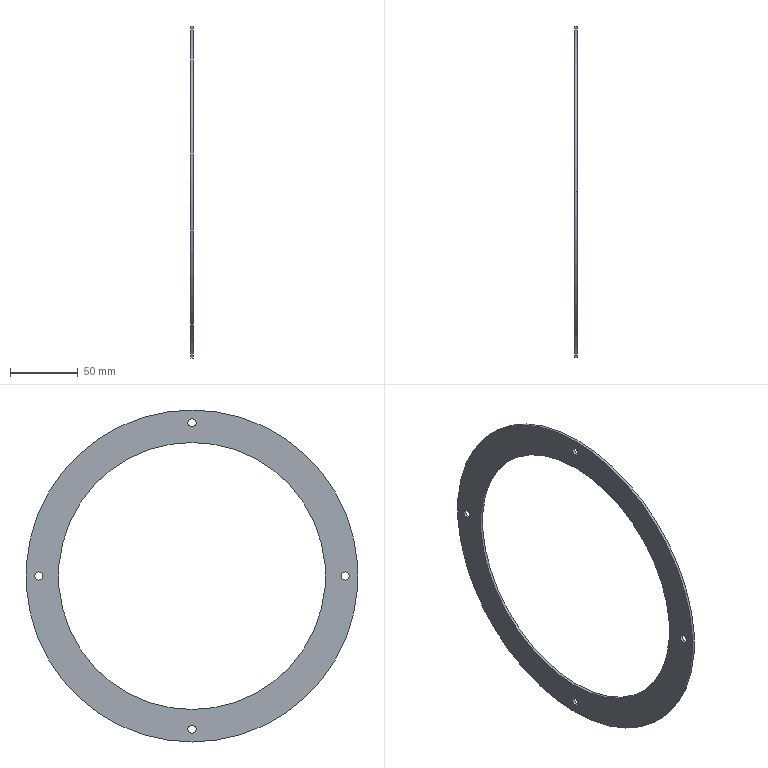Component | SolidWorks | RoundBaffle-1 | 1 solid | 14 faces | box 2 x 245 x 245 mm | volume 33100 mm3 | cylinder 12 | plane 2 | commonest cylinder face diameters 6 x8 197 x2 245 x2
build123d program:
from build123d import *

# Parameters (mm, degrees)
SKETCH1_R           = 122.5
SKETCH1_R_2         = 98.5
BOSS_EXTRUDE1_DEPTH = 2
SKETCH2_R           = 3
CUT_EXTRUDE1_DEPTH  = 10
CIRPATTERN1_COUNT   = 4


with BuildPart() as part:
    # Sketch1 → Boss-Extrude1 (new body)
    with BuildSketch(Plane.XY):
        Circle(SKETCH1_R)
        Circle(SKETCH1_R_2, mode=Mode.SUBTRACT)
    extrude(amount=BOSS_EXTRUDE1_DEPTH)

    # Sketch2 → Cut-Extrude1 (cut)
    with BuildSketch(Plane.XY.offset(2)):
        with Locations((0, 113)):
            Circle(SKETCH2_R)
    cut_extrude1 = extrude(amount=-CUT_EXTRUDE1_DEPTH, mode=Mode.SUBTRACT)

    # CirPattern1: Cut-Extrude1 ×4 about axis
    cirpattern1_axis = Axis((0, 0, 0), (0, 0, 1))
    for i in range(1, CIRPATTERN1_COUNT):
        add(cut_extrude1.rotate(cirpattern1_axis, i * 360 / CIRPATTERN1_COUNT), mode=Mode.SUBTRACT)


solid = part.part

# Placed as in the assembly
solid = solid.moved(Location((-292.55, -77.904, 57.481), (0, 90, 0)))
STEP:
#1=COLOUR_RGB('',0.7922,0.8196,0.9333);
#2=FILL_AREA_STYLE_COLOUR('',#1);
#3=FILL_AREA_STYLE('',(#2));
#4=SURFACE_STYLE_FILL_AREA(#3);
#5=SURFACE_SIDE_STYLE('',(#4));
#6=SURFACE_STYLE_USAGE(.BOTH.,#5);
#7=PRESENTATION_STYLE_ASSIGNMENT((#6));
#8=CARTESIAN_POINT('',(-11.439,-3.067,6.594));
#9=VERTEX_POINT('',#8);
#10=CARTESIAN_POINT('',(-11.439,-3.067,6.83));
#11=VERTEX_POINT('',#10);
#12=CARTESIAN_POINT('',(-11.439,-3.067,6.712));
#13=DIRECTION('',(-1.,0.,0.));
#14=DIRECTION('',(0.,0.,1.));
#15=AXIS2_PLACEMENT_3D('',#12,#13,#14);
#16=CIRCLE('',#15,0.1181);
#17=EDGE_CURVE('',#9,#11,#16,.T.);
#18=ORIENTED_EDGE('',*,*,#17,.F.);
#19=CARTESIAN_POINT('',(-11.518,-3.067,6.594));
#20=VERTEX_POINT('',#19);
#21=CARTESIAN_POINT('',(-11.124,-3.067,6.594));
#22=DIRECTION('',(-1.,0.,0.));
#23=VECTOR('',#22,39.37);
#24=LINE('',#21,#23);
#25=EDGE_CURVE('',#9,#20,#24,.T.);
#26=ORIENTED_EDGE('',*,*,#25,.T.);
#27=CARTESIAN_POINT('',(-11.518,-3.067,6.83));
#28=VERTEX_POINT('',#27);
#29=CARTESIAN_POINT('',(-11.518,-3.067,6.712));
#30=DIRECTION('',(-1.,0.,0.));
#31=DIRECTION('',(0.,-1.,0.));
#32=AXIS2_PLACEMENT_3D('',#29,#30,#31);
#33=CIRCLE('',#32,0.1181);
#34=EDGE_CURVE('',#20,#28,#33,.T.);
#35=ORIENTED_EDGE('',*,*,#34,.T.);
#36=CARTESIAN_POINT('',(-11.124,-3.067,6.83));
#37=DIRECTION('',(-1.,0.,0.));
#38=VECTOR('',#37,39.37);
#39=LINE('',#36,#38);
#40=EDGE_CURVE('',#11,#28,#39,.T.);
#41=ORIENTED_EDGE('',*,*,#40,.F.);
#42=EDGE_LOOP('',(#18,#26,#35,#41));
#43=FACE_OUTER_BOUND('',#42,.T.);
#44=CARTESIAN_POINT('',(-11.124,-3.067,6.712));
#45=DIRECTION('',(-1.,0.,0.));
#46=DIRECTION('',(0.,0.,1.));
#47=AXIS2_PLACEMENT_3D('',#44,#45,#46);
#48=CYLINDRICAL_SURFACE('',#47,0.1181);
#49=ADVANCED_FACE('',(#43),#48,.F.);
#50=CARTESIAN_POINT('',(-11.439,-7.516,2.145));
#51=VERTEX_POINT('',#50);
#52=CARTESIAN_POINT('',(-11.439,-7.516,2.381));
#53=VERTEX_POINT('',#52);
#54=CARTESIAN_POINT('',(-11.439,-7.516,2.263));
#55=DIRECTION('',(-1.,0.,0.));
#56=DIRECTION('',(0.,0.,1.));
#57=AXIS2_PLACEMENT_3D('',#54,#55,#56);
#58=CIRCLE('',#57,0.1181);
#59=EDGE_CURVE('',#51,#53,#58,.T.);
#60=ORIENTED_EDGE('',*,*,#59,.F.);
#61=CARTESIAN_POINT('',(-11.518,-7.516,2.145));
#62=VERTEX_POINT('',#61);
#63=CARTESIAN_POINT('',(-11.124,-7.516,2.145));
#64=DIRECTION('',(-1.,0.,0.));
#65=VECTOR('',#64,39.37);
#66=LINE('',#63,#65);
#67=EDGE_CURVE('',#51,#62,#66,.T.);
#68=ORIENTED_EDGE('',*,*,#67,.T.);
#69=CARTESIAN_POINT('',(-11.518,-7.516,2.381));
#70=VERTEX_POINT('',#69);
#71=CARTESIAN_POINT('',(-11.518,-7.516,2.263));
#72=DIRECTION('',(-1.,0.,0.));
#73=DIRECTION('',(0.,0.,-1.));
#74=AXIS2_PLACEMENT_3D('',#71,#72,#73);
#75=CIRCLE('',#74,0.1181);
#76=EDGE_CURVE('',#62,#70,#75,.T.);
#77=ORIENTED_EDGE('',*,*,#76,.T.);
#78=CARTESIAN_POINT('',(-11.124,-7.516,2.381));
#79=DIRECTION('',(-1.,0.,0.));
#80=VECTOR('',#79,39.37);
#81=LINE('',#78,#80);
#82=EDGE_CURVE('',#53,#70,#81,.T.);
#83=ORIENTED_EDGE('',*,*,#82,.F.);
#84=EDGE_LOOP('',(#60,#68,#77,#83));
#85=FACE_OUTER_BOUND('',#84,.T.);
#86=CARTESIAN_POINT('',(-11.124,-7.516,2.263));
#87=DIRECTION('',(-1.,0.,0.));
#88=DIRECTION('',(0.,0.,1.));
#89=AXIS2_PLACEMENT_3D('',#86,#87,#88);
#90=CYLINDRICAL_SURFACE('',#89,0.1181);
#91=ADVANCED_FACE('',(#85),#90,.F.);
#92=CARTESIAN_POINT('',(-11.439,-3.067,-2.304));
#93=VERTEX_POINT('',#92);
#94=CARTESIAN_POINT('',(-11.439,-3.067,-2.068));
#95=VERTEX_POINT('',#94);
#96=CARTESIAN_POINT('',(-11.439,-3.067,-2.186));
#97=DIRECTION('',(-1.,0.,0.));
#98=DIRECTION('',(0.,0.,1.));
#99=AXIS2_PLACEMENT_3D('',#96,#97,#98);
#100=CIRCLE('',#99,0.1181);
#101=EDGE_CURVE('',#93,#95,#100,.T.);
#102=ORIENTED_EDGE('',*,*,#101,.F.);
#103=CARTESIAN_POINT('',(-11.518,-3.067,-2.304));
#104=VERTEX_POINT('',#103);
#105=CARTESIAN_POINT('',(-11.124,-3.067,-2.304));
#106=DIRECTION('',(-1.,0.,0.));
#107=VECTOR('',#106,39.37);
#108=LINE('',#105,#107);
#109=EDGE_CURVE('',#93,#104,#108,.T.);
#110=ORIENTED_EDGE('',*,*,#109,.T.);
#111=CARTESIAN_POINT('',(-11.518,-3.067,-2.068));
#112=VERTEX_POINT('',#111);
#113=CARTESIAN_POINT('',(-11.518,-3.067,-2.186));
#114=DIRECTION('',(-1.,0.,0.));
#115=DIRECTION('',(0.,1.,-0.));
#116=AXIS2_PLACEMENT_3D('',#113,#114,#115);
#117=CIRCLE('',#116,0.1181);
#118=EDGE_CURVE('',#104,#112,#117,.T.);
#119=ORIENTED_EDGE('',*,*,#118,.T.);
#120=CARTESIAN_POINT('',(-11.124,-3.067,-2.068));
#121=DIRECTION('',(-1.,0.,0.));
#122=VECTOR('',#121,39.37);
#123=LINE('',#120,#122);
#124=EDGE_CURVE('',#95,#112,#123,.T.);
#125=ORIENTED_EDGE('',*,*,#124,.F.);
#126=EDGE_LOOP('',(#102,#110,#119,#125));
#127=FACE_OUTER_BOUND('',#126,.T.);
#128=CARTESIAN_POINT('',(-11.124,-3.067,-2.186));
#129=DIRECTION('',(-1.,0.,0.));
#130=DIRECTION('',(0.,0.,1.));
#131=AXIS2_PLACEMENT_3D('',#128,#129,#130);
#132=CYLINDRICAL_SURFACE('',#131,0.1181);
#133=ADVANCED_FACE('',(#127),#132,.F.);
#134=CARTESIAN_POINT('',(-11.439,1.382,2.145));
#135=VERTEX_POINT('',#134);
#136=CARTESIAN_POINT('',(-11.439,1.382,2.381));
#137=VERTEX_POINT('',#136);
#138=CARTESIAN_POINT('',(-11.439,1.382,2.263));
#139=DIRECTION('',(-1.,0.,0.));
#140=DIRECTION('',(0.,0.,1.));
#141=AXIS2_PLACEMENT_3D('',#138,#139,#140);
#142=CIRCLE('',#141,0.1181);
#143=EDGE_CURVE('',#135,#137,#142,.T.);
#144=ORIENTED_EDGE('',*,*,#143,.F.);
#145=CARTESIAN_POINT('',(-11.518,1.382,2.145));
#146=VERTEX_POINT('',#145);
#147=CARTESIAN_POINT('',(-11.124,1.382,2.145));
#148=DIRECTION('',(-1.,0.,0.));
#149=VECTOR('',#148,39.37);
#150=LINE('',#147,#149);
#151=EDGE_CURVE('',#135,#146,#150,.T.);
#152=ORIENTED_EDGE('',*,*,#151,.T.);
#153=CARTESIAN_POINT('',(-11.518,1.382,2.381));
#154=VERTEX_POINT('',#153);
#155=CARTESIAN_POINT('',(-11.518,1.382,2.263));
#156=DIRECTION('',(-1.,0.,0.));
#157=DIRECTION('',(0.,0.,1.));
#158=AXIS2_PLACEMENT_3D('',#155,#156,#157);
#159=CIRCLE('',#158,0.1181);
#160=EDGE_CURVE('',#146,#154,#159,.T.);
#161=ORIENTED_EDGE('',*,*,#160,.T.);
#162=CARTESIAN_POINT('',(-11.124,1.382,2.381));
#163=DIRECTION('',(-1.,0.,0.));
#164=VECTOR('',#163,39.37);
#165=LINE('',#162,#164);
#166=EDGE_CURVE('',#137,#154,#165,.T.);
#167=ORIENTED_EDGE('',*,*,#166,.F.);
#168=EDGE_LOOP('',(#144,#152,#161,#167));
#169=FACE_OUTER_BOUND('',#168,.T.);
#170=CARTESIAN_POINT('',(-11.124,1.382,2.263));
#171=DIRECTION('',(-1.,0.,0.));
#172=DIRECTION('',(0.,0.,1.));
#173=AXIS2_PLACEMENT_3D('',#170,#171,#172);
#174=CYLINDRICAL_SURFACE('',#173,0.1181);
#175=ADVANCED_FACE('',(#169),#174,.F.);
#176=CARTESIAN_POINT('',(-11.518,-3.067,-1.615));
#177=VERTEX_POINT('',#176);
#178=CARTESIAN_POINT('',(-11.518,-3.067,6.141));
#179=VERTEX_POINT('',#178);
#180=CARTESIAN_POINT('',(-11.518,-3.067,2.263));
#181=DIRECTION('',(-1.,0.,0.));
#182=DIRECTION('',(0.,0.,1.));
#183=AXIS2_PLACEMENT_3D('',#180,#181,#182);
#184=CIRCLE('',#183,3.878);
#185=EDGE_CURVE('',#177,#179,#184,.T.);
#186=ORIENTED_EDGE('',*,*,#185,.T.);
#187=CARTESIAN_POINT('',(-11.439,-3.067,6.141));
#188=VERTEX_POINT('',#187);
#189=CARTESIAN_POINT('',(-11.518,-3.067,6.141));
#190=DIRECTION('',(1.,0.,0.));
#191=VECTOR('',#190,39.37);
#192=LINE('',#189,#191);
#193=EDGE_CURVE('',#179,#188,#192,.T.);
#194=ORIENTED_EDGE('',*,*,#193,.T.);
#195=CARTESIAN_POINT('',(-11.439,-3.067,-1.615));
#196=VERTEX_POINT('',#195);
#197=CARTESIAN_POINT('',(-11.439,-3.067,2.263));
#198=DIRECTION('',(-1.,0.,0.));
#199=DIRECTION('',(0.,0.,1.));
#200=AXIS2_PLACEMENT_3D('',#197,#198,#199);
#201=CIRCLE('',#200,3.878);
#202=EDGE_CURVE('',#196,#188,#201,.T.);
#203=ORIENTED_EDGE('',*,*,#202,.F.);
#204=CARTESIAN_POINT('',(-11.518,-3.067,-1.615));
#205=DIRECTION('',(1.,0.,0.));
#206=VECTOR('',#205,39.37);
#207=LINE('',#204,#206);
#208=EDGE_CURVE('',#177,#196,#207,.T.);
#209=ORIENTED_EDGE('',*,*,#208,.F.);
#210=EDGE_LOOP('',(#186,#194,#203,#209));
#211=FACE_OUTER_BOUND('',#210,.T.);
#212=CARTESIAN_POINT('',(-11.518,-3.067,2.263));
#213=DIRECTION('',(1.,0.,0.));
#214=DIRECTION('',(0.,0.,-1.));
#215=AXIS2_PLACEMENT_3D('',#212,#213,#214);
#216=CYLINDRICAL_SURFACE('',#215,3.878);
#217=ADVANCED_FACE('',(#211),#216,.F.);
#218=CARTESIAN_POINT('',(-11.518,-3.067,7.086));
#219=VERTEX_POINT('',#218);
#220=CARTESIAN_POINT('',(-11.518,-3.067,-2.56));
#221=VERTEX_POINT('',#220);
#222=CARTESIAN_POINT('',(-11.518,-3.067,2.263));
#223=DIRECTION('',(-1.,0.,0.));
#224=DIRECTION('',(0.,0.,1.));
#225=AXIS2_PLACEMENT_3D('',#222,#223,#224);
#226=CIRCLE('',#225,4.823);
#227=EDGE_CURVE('',#219,#221,#226,.T.);
#228=ORIENTED_EDGE('',*,*,#227,.F.);
#229=CARTESIAN_POINT('',(-11.439,-3.067,7.086));
#230=VERTEX_POINT('',#229);
#231=CARTESIAN_POINT('',(-11.518,-3.067,7.086));
#232=DIRECTION('',(1.,0.,0.));
#233=VECTOR('',#232,39.37);
#234=LINE('',#231,#233);
#235=EDGE_CURVE('',#219,#230,#234,.T.);
#236=ORIENTED_EDGE('',*,*,#235,.T.);
#237=CARTESIAN_POINT('',(-11.439,-3.067,-2.56));
#238=VERTEX_POINT('',#237);
#239=CARTESIAN_POINT('',(-11.439,-3.067,2.263));
#240=DIRECTION('',(-1.,0.,0.));
#241=DIRECTION('',(0.,0.,1.));
#242=AXIS2_PLACEMENT_3D('',#239,#240,#241);
#243=CIRCLE('',#242,4.823);
#244=EDGE_CURVE('',#230,#238,#243,.T.);
#245=ORIENTED_EDGE('',*,*,#244,.T.);
#246=CARTESIAN_POINT('',(-11.518,-3.067,-2.56));
#247=DIRECTION('',(1.,0.,0.));
#248=VECTOR('',#247,39.37);
#249=LINE('',#246,#248);
#250=EDGE_CURVE('',#221,#238,#249,.T.);
#251=ORIENTED_EDGE('',*,*,#250,.F.);
#252=EDGE_LOOP('',(#228,#236,#245,#251));
#253=FACE_OUTER_BOUND('',#252,.T.);
#254=CARTESIAN_POINT('',(-11.518,-3.067,2.263));
#255=DIRECTION('',(1.,0.,0.));
#256=DIRECTION('',(0.,0.,-1.));
#257=AXIS2_PLACEMENT_3D('',#254,#255,#256);
#258=CYLINDRICAL_SURFACE('',#257,4.823);
#259=ADVANCED_FACE('',(#253),#258,.T.);
#260=CARTESIAN_POINT('',(-11.518,-3.067,6.712));
#261=DIRECTION('',(-1.,0.,0.));
#262=DIRECTION('',(0.,-1.,0.));
#263=AXIS2_PLACEMENT_3D('',#260,#261,#262);
#264=CIRCLE('',#263,0.1181);
#265=EDGE_CURVE('',#28,#20,#264,.T.);
#266=ORIENTED_EDGE('',*,*,#265,.F.);
#267=ORIENTED_EDGE('',*,*,#34,.F.);
#268=EDGE_LOOP('',(#266,#267));
#269=FACE_BOUND('',#268,.T.);
#270=CARTESIAN_POINT('',(-11.518,-7.516,2.263));
#271=DIRECTION('',(-1.,0.,0.));
#272=DIRECTION('',(0.,0.,-1.));
#273=AXIS2_PLACEMENT_3D('',#270,#271,#272);
#274=CIRCLE('',#273,0.1181);
#275=EDGE_CURVE('',#70,#62,#274,.T.);
#276=ORIENTED_EDGE('',*,*,#275,.F.);
#277=ORIENTED_EDGE('',*,*,#76,.F.);
#278=EDGE_LOOP('',(#276,#277));
#279=FACE_BOUND('',#278,.T.);
#280=CARTESIAN_POINT('',(-11.518,-3.067,-2.186));
#281=DIRECTION('',(-1.,0.,0.));
#282=DIRECTION('',(0.,1.,-0.));
#283=AXIS2_PLACEMENT_3D('',#280,#281,#282);
#284=CIRCLE('',#283,0.1181);
#285=EDGE_CURVE('',#112,#104,#284,.T.);
#286=ORIENTED_EDGE('',*,*,#285,.F.);
#287=ORIENTED_EDGE('',*,*,#118,.F.);
#288=EDGE_LOOP('',(#286,#287));
#289=FACE_BOUND('',#288,.T.);
#290=CARTESIAN_POINT('',(-11.518,1.382,2.263));
#291=DIRECTION('',(-1.,0.,0.));
#292=DIRECTION('',(0.,0.,1.));
#293=AXIS2_PLACEMENT_3D('',#290,#291,#292);
#294=CIRCLE('',#293,0.1181);
#295=EDGE_CURVE('',#154,#146,#294,.T.);
#296=ORIENTED_EDGE('',*,*,#295,.F.);
#297=ORIENTED_EDGE('',*,*,#160,.F.);
#298=EDGE_LOOP('',(#296,#297));
#299=FACE_BOUND('',#298,.T.);
#300=CARTESIAN_POINT('',(-11.518,-3.067,2.263));
#301=DIRECTION('',(-1.,0.,0.));
#302=DIRECTION('',(0.,0.,1.));
#303=AXIS2_PLACEMENT_3D('',#300,#301,#302);
#304=CIRCLE('',#303,4.823);
#305=EDGE_CURVE('',#221,#219,#304,.T.);
#306=ORIENTED_EDGE('',*,*,#305,.T.);
#307=ORIENTED_EDGE('',*,*,#227,.T.);
#308=EDGE_LOOP('',(#306,#307));
#309=FACE_OUTER_BOUND('',#308,.T.);
#310=ORIENTED_EDGE('',*,*,#185,.F.);
#311=CARTESIAN_POINT('',(-11.518,-3.067,2.263));
#312=DIRECTION('',(-1.,0.,0.));
#313=DIRECTION('',(0.,0.,1.));
#314=AXIS2_PLACEMENT_3D('',#311,#312,#313);
#315=CIRCLE('',#314,3.878);
#316=EDGE_CURVE('',#179,#177,#315,.T.);
#317=ORIENTED_EDGE('',*,*,#316,.F.);
#318=EDGE_LOOP('',(#310,#317));
#319=FACE_BOUND('',#318,.T.);
#320=CARTESIAN_POINT('',(-11.518,-3.067,2.263));
#321=DIRECTION('',(-1.,0.,0.));
#322=DIRECTION('',(0.,0.,1.));
#323=AXIS2_PLACEMENT_3D('',#320,#321,#322);
#324=PLANE('',#323);
#325=ADVANCED_FACE('',(#269,#279,#289,#299,#309,#319),#324,.T.);
#326=CARTESIAN_POINT('',(-11.439,-3.067,6.712));
#327=DIRECTION('',(-1.,0.,0.));
#328=DIRECTION('',(0.,0.,1.));
#329=AXIS2_PLACEMENT_3D('',#326,#327,#328);
#330=CIRCLE('',#329,0.1181);
#331=EDGE_CURVE('',#11,#9,#330,.T.);
#332=ORIENTED_EDGE('',*,*,#331,.T.);
#333=ORIENTED_EDGE('',*,*,#17,.T.);
#334=EDGE_LOOP('',(#332,#333));
#335=FACE_BOUND('',#334,.T.);
#336=CARTESIAN_POINT('',(-11.439,-7.516,2.263));
#337=DIRECTION('',(-1.,0.,0.));
#338=DIRECTION('',(0.,0.,1.));
#339=AXIS2_PLACEMENT_3D('',#336,#337,#338);
#340=CIRCLE('',#339,0.1181);
#341=EDGE_CURVE('',#53,#51,#340,.T.);
#342=ORIENTED_EDGE('',*,*,#341,.T.);
#343=ORIENTED_EDGE('',*,*,#59,.T.);
#344=EDGE_LOOP('',(#342,#343));
#345=FACE_BOUND('',#344,.T.);
#346=CARTESIAN_POINT('',(-11.439,-3.067,-2.186));
#347=DIRECTION('',(-1.,0.,0.));
#348=DIRECTION('',(0.,0.,1.));
#349=AXIS2_PLACEMENT_3D('',#346,#347,#348);
#350=CIRCLE('',#349,0.1181);
#351=EDGE_CURVE('',#95,#93,#350,.T.);
#352=ORIENTED_EDGE('',*,*,#351,.T.);
#353=ORIENTED_EDGE('',*,*,#101,.T.);
#354=EDGE_LOOP('',(#352,#353));
#355=FACE_BOUND('',#354,.T.);
#356=CARTESIAN_POINT('',(-11.439,1.382,2.263));
#357=DIRECTION('',(-1.,0.,0.));
#358=DIRECTION('',(0.,0.,1.));
#359=AXIS2_PLACEMENT_3D('',#356,#357,#358);
#360=CIRCLE('',#359,0.1181);
#361=EDGE_CURVE('',#137,#135,#360,.T.);
#362=ORIENTED_EDGE('',*,*,#361,.T.);
#363=ORIENTED_EDGE('',*,*,#143,.T.);
#364=EDGE_LOOP('',(#362,#363));
#365=FACE_BOUND('',#364,.T.);
#366=CARTESIAN_POINT('',(-11.439,-3.067,2.263));
#367=DIRECTION('',(-1.,0.,0.));
#368=DIRECTION('',(0.,0.,1.));
#369=AXIS2_PLACEMENT_3D('',#366,#367,#368);
#370=CIRCLE('',#369,4.823);
#371=EDGE_CURVE('',#238,#230,#370,.T.);
#372=ORIENTED_EDGE('',*,*,#371,.F.);
#373=ORIENTED_EDGE('',*,*,#244,.F.);
#374=EDGE_LOOP('',(#372,#373));
#375=FACE_OUTER_BOUND('',#374,.T.);
#376=ORIENTED_EDGE('',*,*,#202,.T.);
#377=CARTESIAN_POINT('',(-11.439,-3.067,2.263));
#378=DIRECTION('',(-1.,0.,0.));
#379=DIRECTION('',(0.,0.,1.));
#380=AXIS2_PLACEMENT_3D('',#377,#378,#379);
#381=CIRCLE('',#380,3.878);
#382=EDGE_CURVE('',#188,#196,#381,.T.);
#383=ORIENTED_EDGE('',*,*,#382,.T.);
#384=EDGE_LOOP('',(#376,#383));
#385=FACE_BOUND('',#384,.T.);
#386=CARTESIAN_POINT('',(-11.439,-3.067,2.263));
#387=DIRECTION('',(-1.,0.,0.));
#388=DIRECTION('',(0.,0.,1.));
#389=AXIS2_PLACEMENT_3D('',#386,#387,#388);
#390=PLANE('',#389);
#391=ADVANCED_FACE('',(#335,#345,#355,#365,#375,#385),#390,.F.);
#392=ORIENTED_EDGE('',*,*,#235,.F.);
#393=ORIENTED_EDGE('',*,*,#305,.F.);
#394=ORIENTED_EDGE('',*,*,#250,.T.);
#395=ORIENTED_EDGE('',*,*,#371,.T.);
#396=EDGE_LOOP('',(#392,#393,#394,#395));
#397=FACE_OUTER_BOUND('',#396,.T.);
#398=CARTESIAN_POINT('',(-11.518,-3.067,2.263));
#399=DIRECTION('',(1.,0.,0.));
#400=DIRECTION('',(0.,0.,-1.));
#401=AXIS2_PLACEMENT_3D('',#398,#399,#400);
#402=CYLINDRICAL_SURFACE('',#401,4.823);
#403=ADVANCED_FACE('',(#397),#402,.T.);
#404=ORIENTED_EDGE('',*,*,#193,.F.);
#405=ORIENTED_EDGE('',*,*,#316,.T.);
#406=ORIENTED_EDGE('',*,*,#208,.T.);
#407=ORIENTED_EDGE('',*,*,#382,.F.);
#408=EDGE_LOOP('',(#404,#405,#406,#407));
#409=FACE_OUTER_BOUND('',#408,.T.);
#410=CARTESIAN_POINT('',(-11.518,-3.067,2.263));
#411=DIRECTION('',(1.,0.,0.));
#412=DIRECTION('',(0.,0.,-1.));
#413=AXIS2_PLACEMENT_3D('',#410,#411,#412);
#414=CYLINDRICAL_SURFACE('',#413,3.878);
#415=ADVANCED_FACE('',(#409),#414,.F.);
#416=ORIENTED_EDGE('',*,*,#151,.F.);
#417=ORIENTED_EDGE('',*,*,#361,.F.);
#418=ORIENTED_EDGE('',*,*,#166,.T.);
#419=ORIENTED_EDGE('',*,*,#295,.T.);
#420=EDGE_LOOP('',(#416,#417,#418,#419));
#421=FACE_OUTER_BOUND('',#420,.T.);
#422=CARTESIAN_POINT('',(-11.124,1.382,2.263));
#423=DIRECTION('',(-1.,0.,0.));
#424=DIRECTION('',(0.,0.,1.));
#425=AXIS2_PLACEMENT_3D('',#422,#423,#424);
#426=CYLINDRICAL_SURFACE('',#425,0.1181);
#427=ADVANCED_FACE('',(#421),#426,.F.);
#428=ORIENTED_EDGE('',*,*,#109,.F.);
#429=ORIENTED_EDGE('',*,*,#351,.F.);
#430=ORIENTED_EDGE('',*,*,#124,.T.);
#431=ORIENTED_EDGE('',*,*,#285,.T.);
#432=EDGE_LOOP('',(#428,#429,#430,#431));
#433=FACE_OUTER_BOUND('',#432,.T.);
#434=CARTESIAN_POINT('',(-11.124,-3.067,-2.186));
#435=DIRECTION('',(-1.,0.,0.));
#436=DIRECTION('',(0.,0.,1.));
#437=AXIS2_PLACEMENT_3D('',#434,#435,#436);
#438=CYLINDRICAL_SURFACE('',#437,0.1181);
#439=ADVANCED_FACE('',(#433),#438,.F.);
#440=ORIENTED_EDGE('',*,*,#67,.F.);
#441=ORIENTED_EDGE('',*,*,#341,.F.);
#442=ORIENTED_EDGE('',*,*,#82,.T.);
#443=ORIENTED_EDGE('',*,*,#275,.T.);
#444=EDGE_LOOP('',(#440,#441,#442,#443));
#445=FACE_OUTER_BOUND('',#444,.T.);
#446=CARTESIAN_POINT('',(-11.124,-7.516,2.263));
#447=DIRECTION('',(-1.,0.,0.));
#448=DIRECTION('',(0.,0.,1.));
#449=AXIS2_PLACEMENT_3D('',#446,#447,#448);
#450=CYLINDRICAL_SURFACE('',#449,0.1181);
#451=ADVANCED_FACE('',(#445),#450,.F.);
#452=ORIENTED_EDGE('',*,*,#25,.F.);
#453=ORIENTED_EDGE('',*,*,#331,.F.);
#454=ORIENTED_EDGE('',*,*,#40,.T.);
#455=ORIENTED_EDGE('',*,*,#265,.T.);
#456=EDGE_LOOP('',(#452,#453,#454,#455));
#457=FACE_OUTER_BOUND('',#456,.T.);
#458=CARTESIAN_POINT('',(-11.124,-3.067,6.712));
#459=DIRECTION('',(-1.,0.,0.));
#460=DIRECTION('',(0.,0.,1.));
#461=AXIS2_PLACEMENT_3D('',#458,#459,#460);
#462=CYLINDRICAL_SURFACE('',#461,0.1181);
#463=ADVANCED_FACE('',(#457),#462,.F.);
#464=CLOSED_SHELL('',(#49,#91,#133,#175,#217,#259,#325,#391,#403,#415,#427,#439,#451,#463));
#465=MANIFOLD_SOLID_BREP('',#464);
#466=STYLED_ITEM('',(#7),#465);
#467=(LENGTH_UNIT()NAMED_UNIT(*)SI_UNIT($,.METRE.));
#468=LENGTH_MEASURE_WITH_UNIT(LENGTH_MEASURE(0.0254),#467);
#469=DIMENSIONAL_EXPONENTS(1.,0.,0.,0.,0.,0.,0.);
#470=(CONVERSION_BASED_UNIT('',#468)LENGTH_UNIT()NAMED_UNIT(#469));
#471=UNCERTAINTY_MEASURE_WITH_UNIT(LENGTH_MEASURE(0.00001),#470,'','');
#472=(NAMED_UNIT(*)PLANE_ANGLE_UNIT()SI_UNIT($,.RADIAN.));
#473=(NAMED_UNIT(*)SI_UNIT($,.STERADIAN.)SOLID_ANGLE_UNIT());
#474=(GEOMETRIC_REPRESENTATION_CONTEXT(3)GLOBAL_UNCERTAINTY_ASSIGNED_CONTEXT((#471))GLOBAL_UNIT_ASSIGNED_CONTEXT((#470,#472,#473))REPRESENTATION_CONTEXT('',''));
#475=MECHANICAL_DESIGN_GEOMETRIC_PRESENTATION_REPRESENTATION('',(#466),#474);
#476=PRESENTATION_LAYER_ASSIGNMENT('','',(#466));
#477=CARTESIAN_POINT('',(0.,0.,0.));
#478=DIRECTION('',(0.,0.,1.));
#479=DIRECTION('',(1.,0.,0.));
#480=AXIS2_PLACEMENT_3D('',#477,#478,#479);
#481=(LENGTH_UNIT()NAMED_UNIT(*)SI_UNIT($,.METRE.));
#482=LENGTH_MEASURE_WITH_UNIT(LENGTH_MEASURE(0.0254),#481);
#483=DIMENSIONAL_EXPONENTS(1.,0.,0.,0.,0.,0.,0.);
#484=(CONVERSION_BASED_UNIT('',#482)LENGTH_UNIT()NAMED_UNIT(#483));
#485=UNCERTAINTY_MEASURE_WITH_UNIT(LENGTH_MEASURE(0.00001),#484,'','');
#486=(NAMED_UNIT(*)PLANE_ANGLE_UNIT()SI_UNIT($,.RADIAN.));
#487=(NAMED_UNIT(*)SI_UNIT($,.STERADIAN.)SOLID_ANGLE_UNIT());
#488=(GEOMETRIC_REPRESENTATION_CONTEXT(3)GLOBAL_UNCERTAINTY_ASSIGNED_CONTEXT((#485))GLOBAL_UNIT_ASSIGNED_CONTEXT((#484,#486,#487))REPRESENTATION_CONTEXT('',''));
#489=ADVANCED_BREP_SHAPE_REPRESENTATION('',(#465,#480),#488);